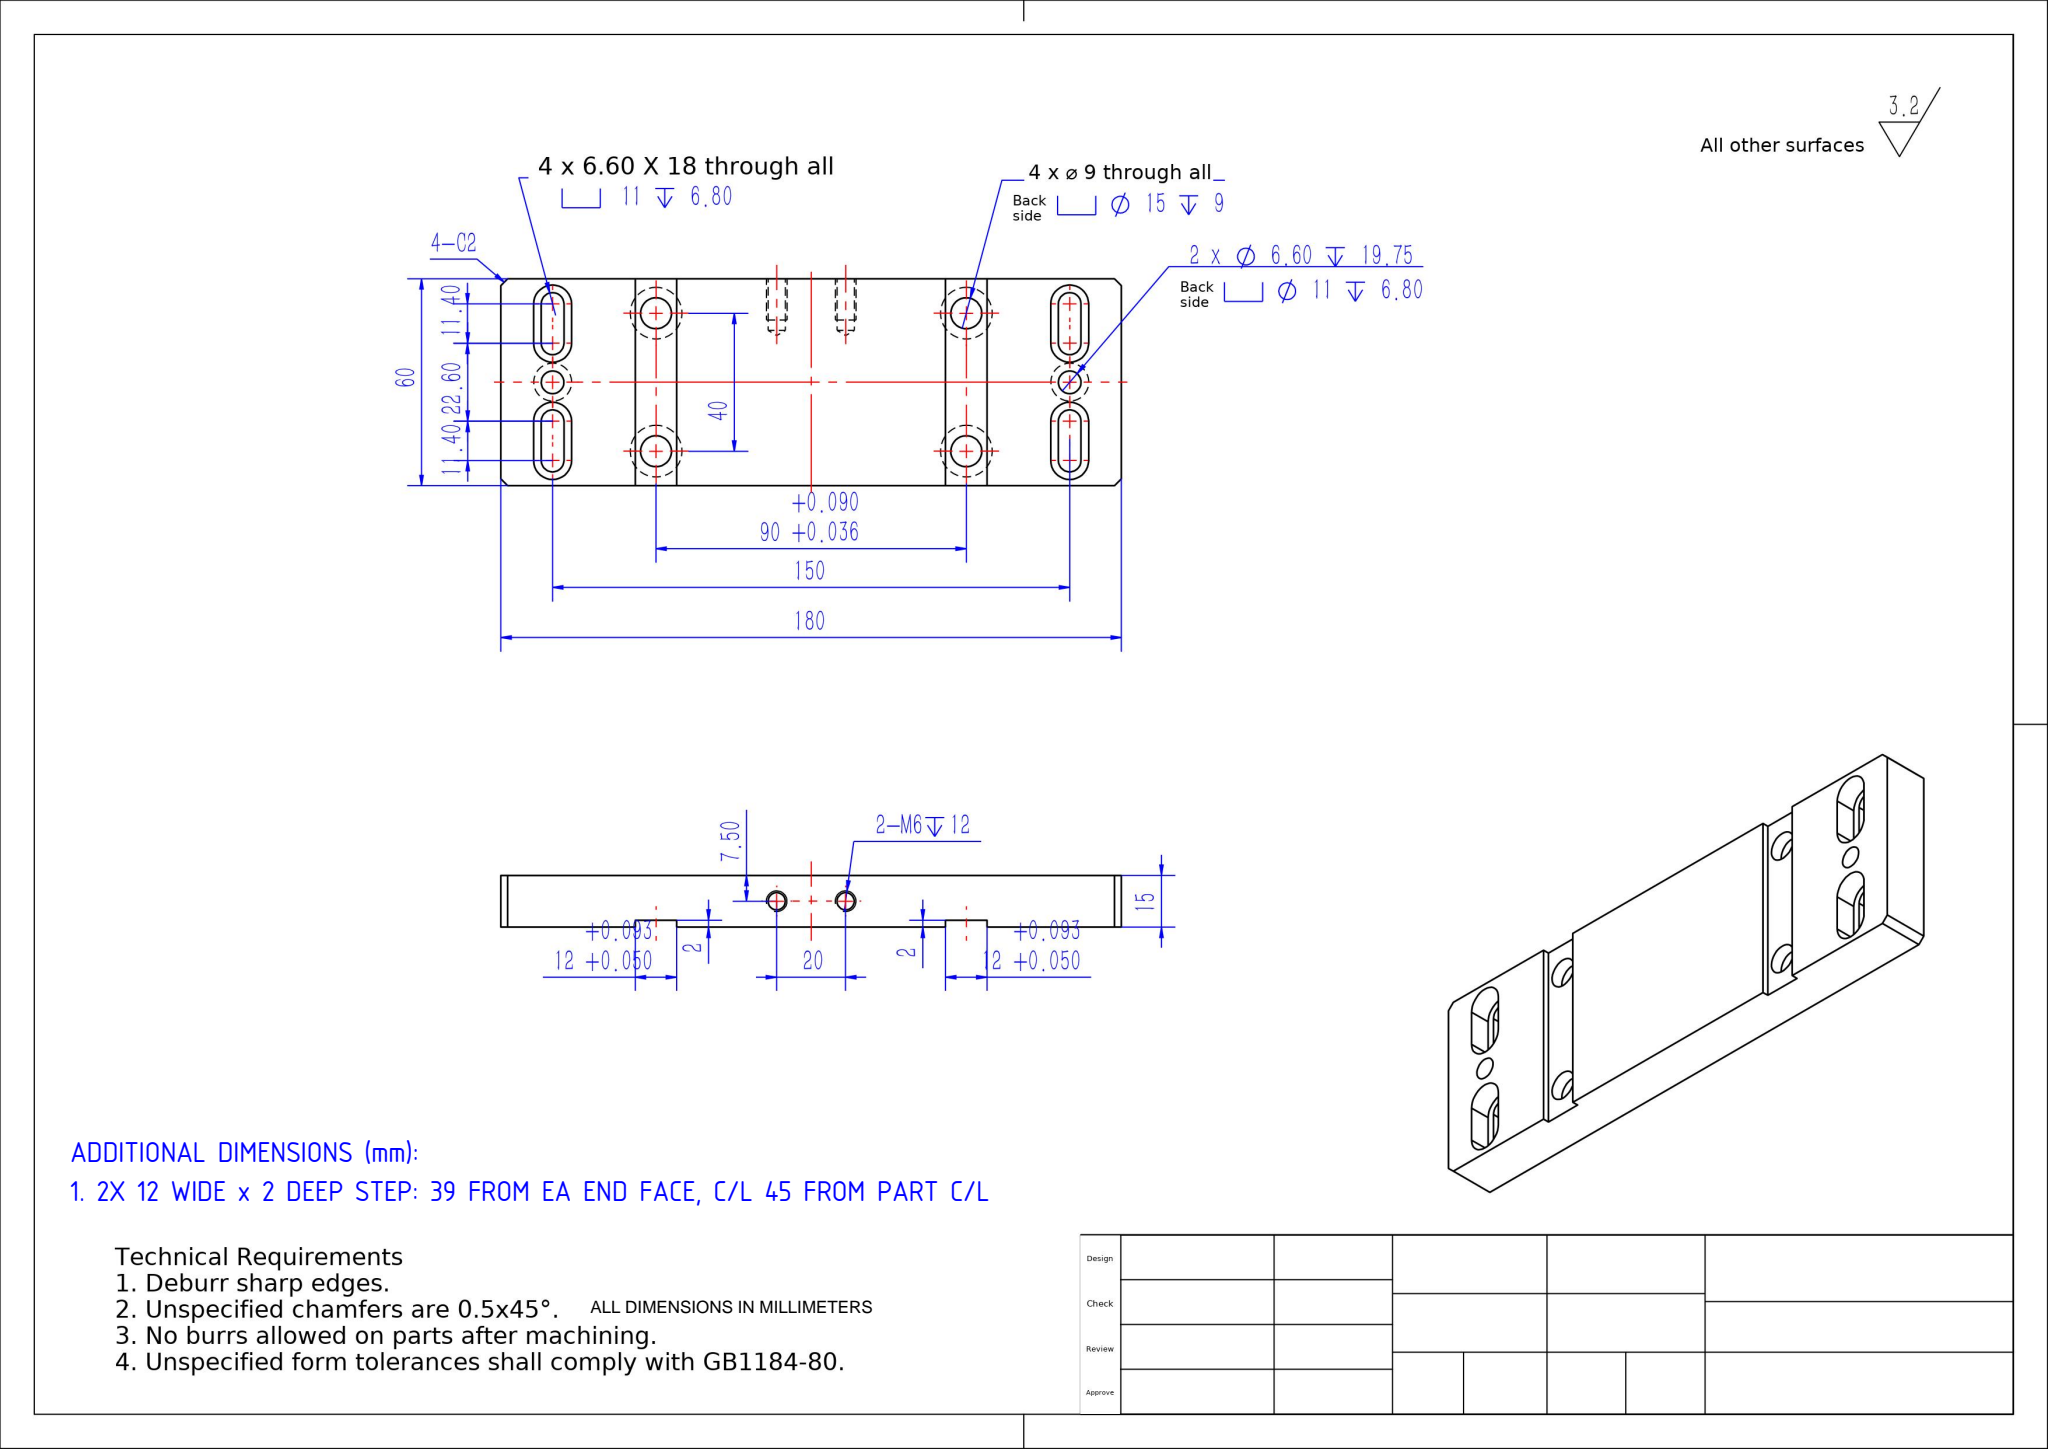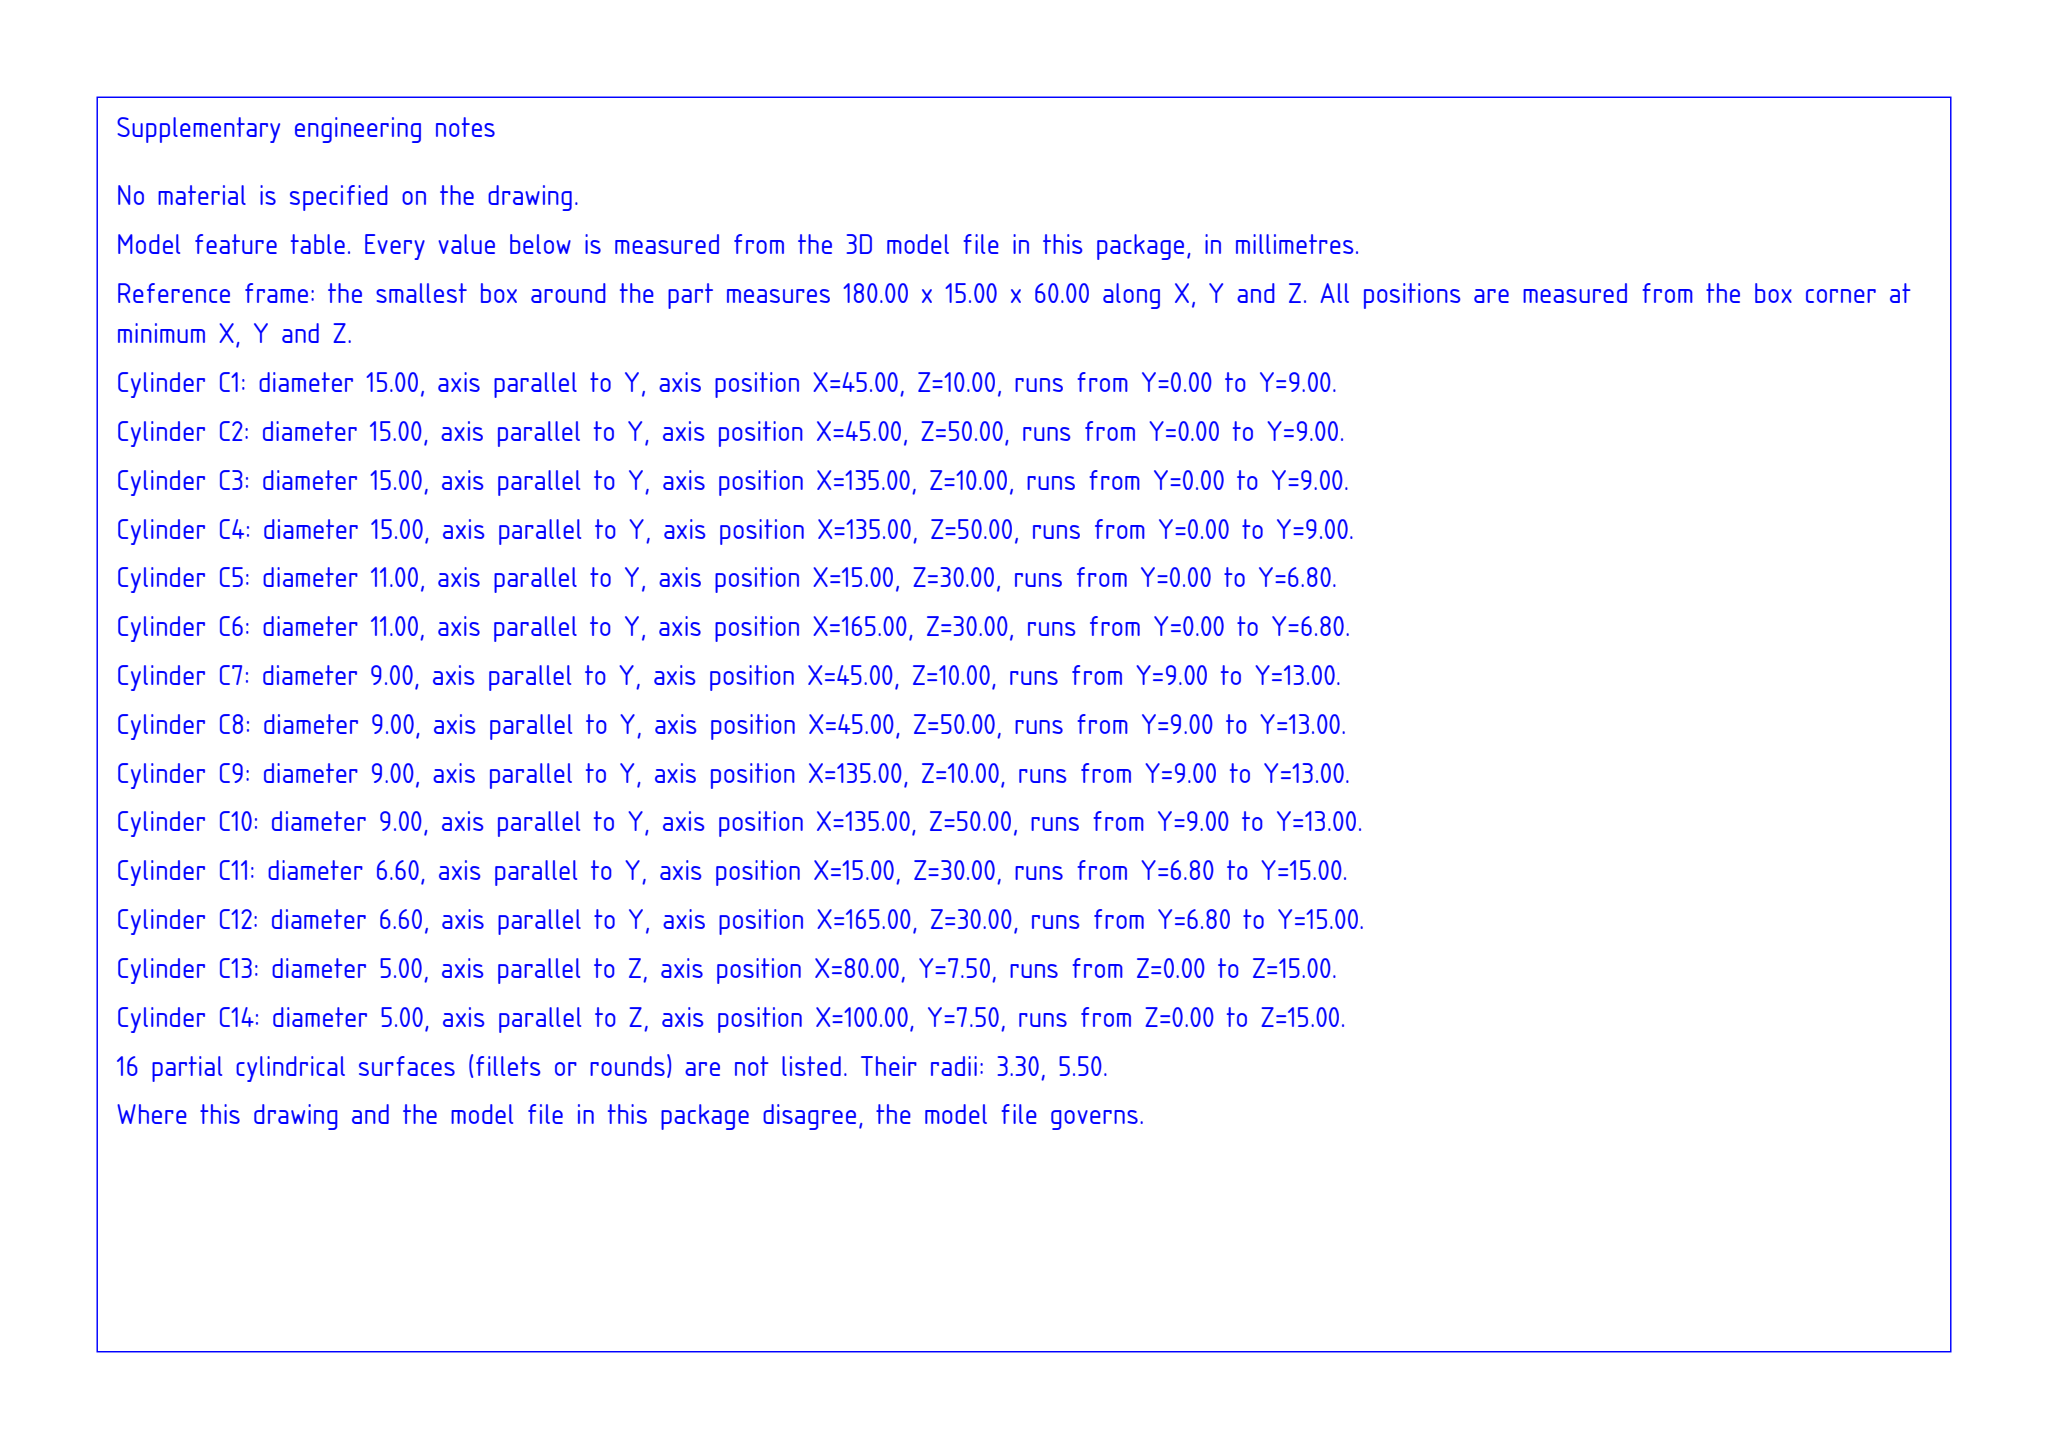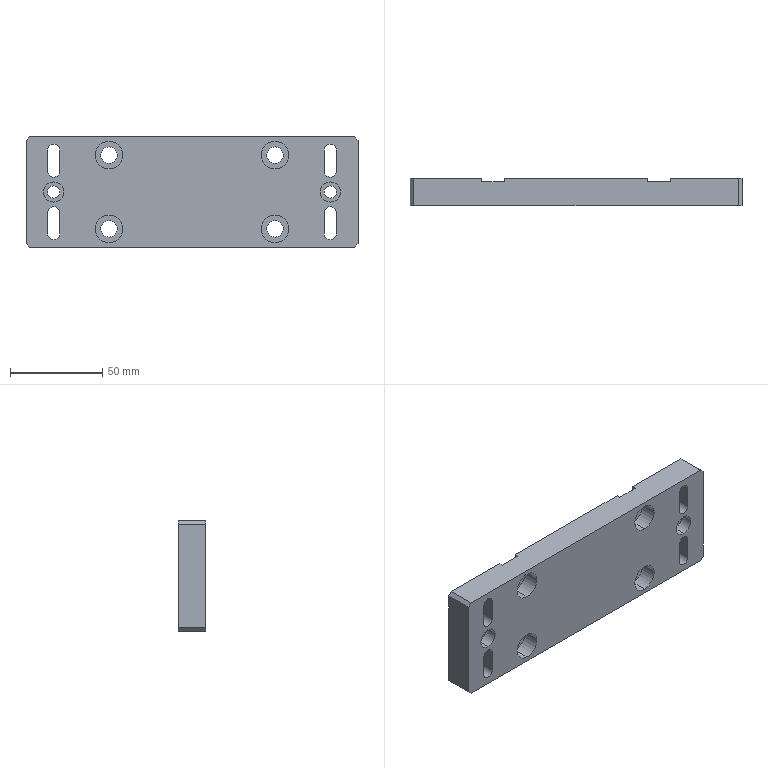Part | SolidWorks | mm | 1 solid | 100 faces | box 180 x 15 x 60 mm | volume 139572 mm3 | cylinder 52 | plane 44 | cone 4 | commonest cylinder face diameters 11 x16 6.6 x16 15 x8 9 x8 5 x4